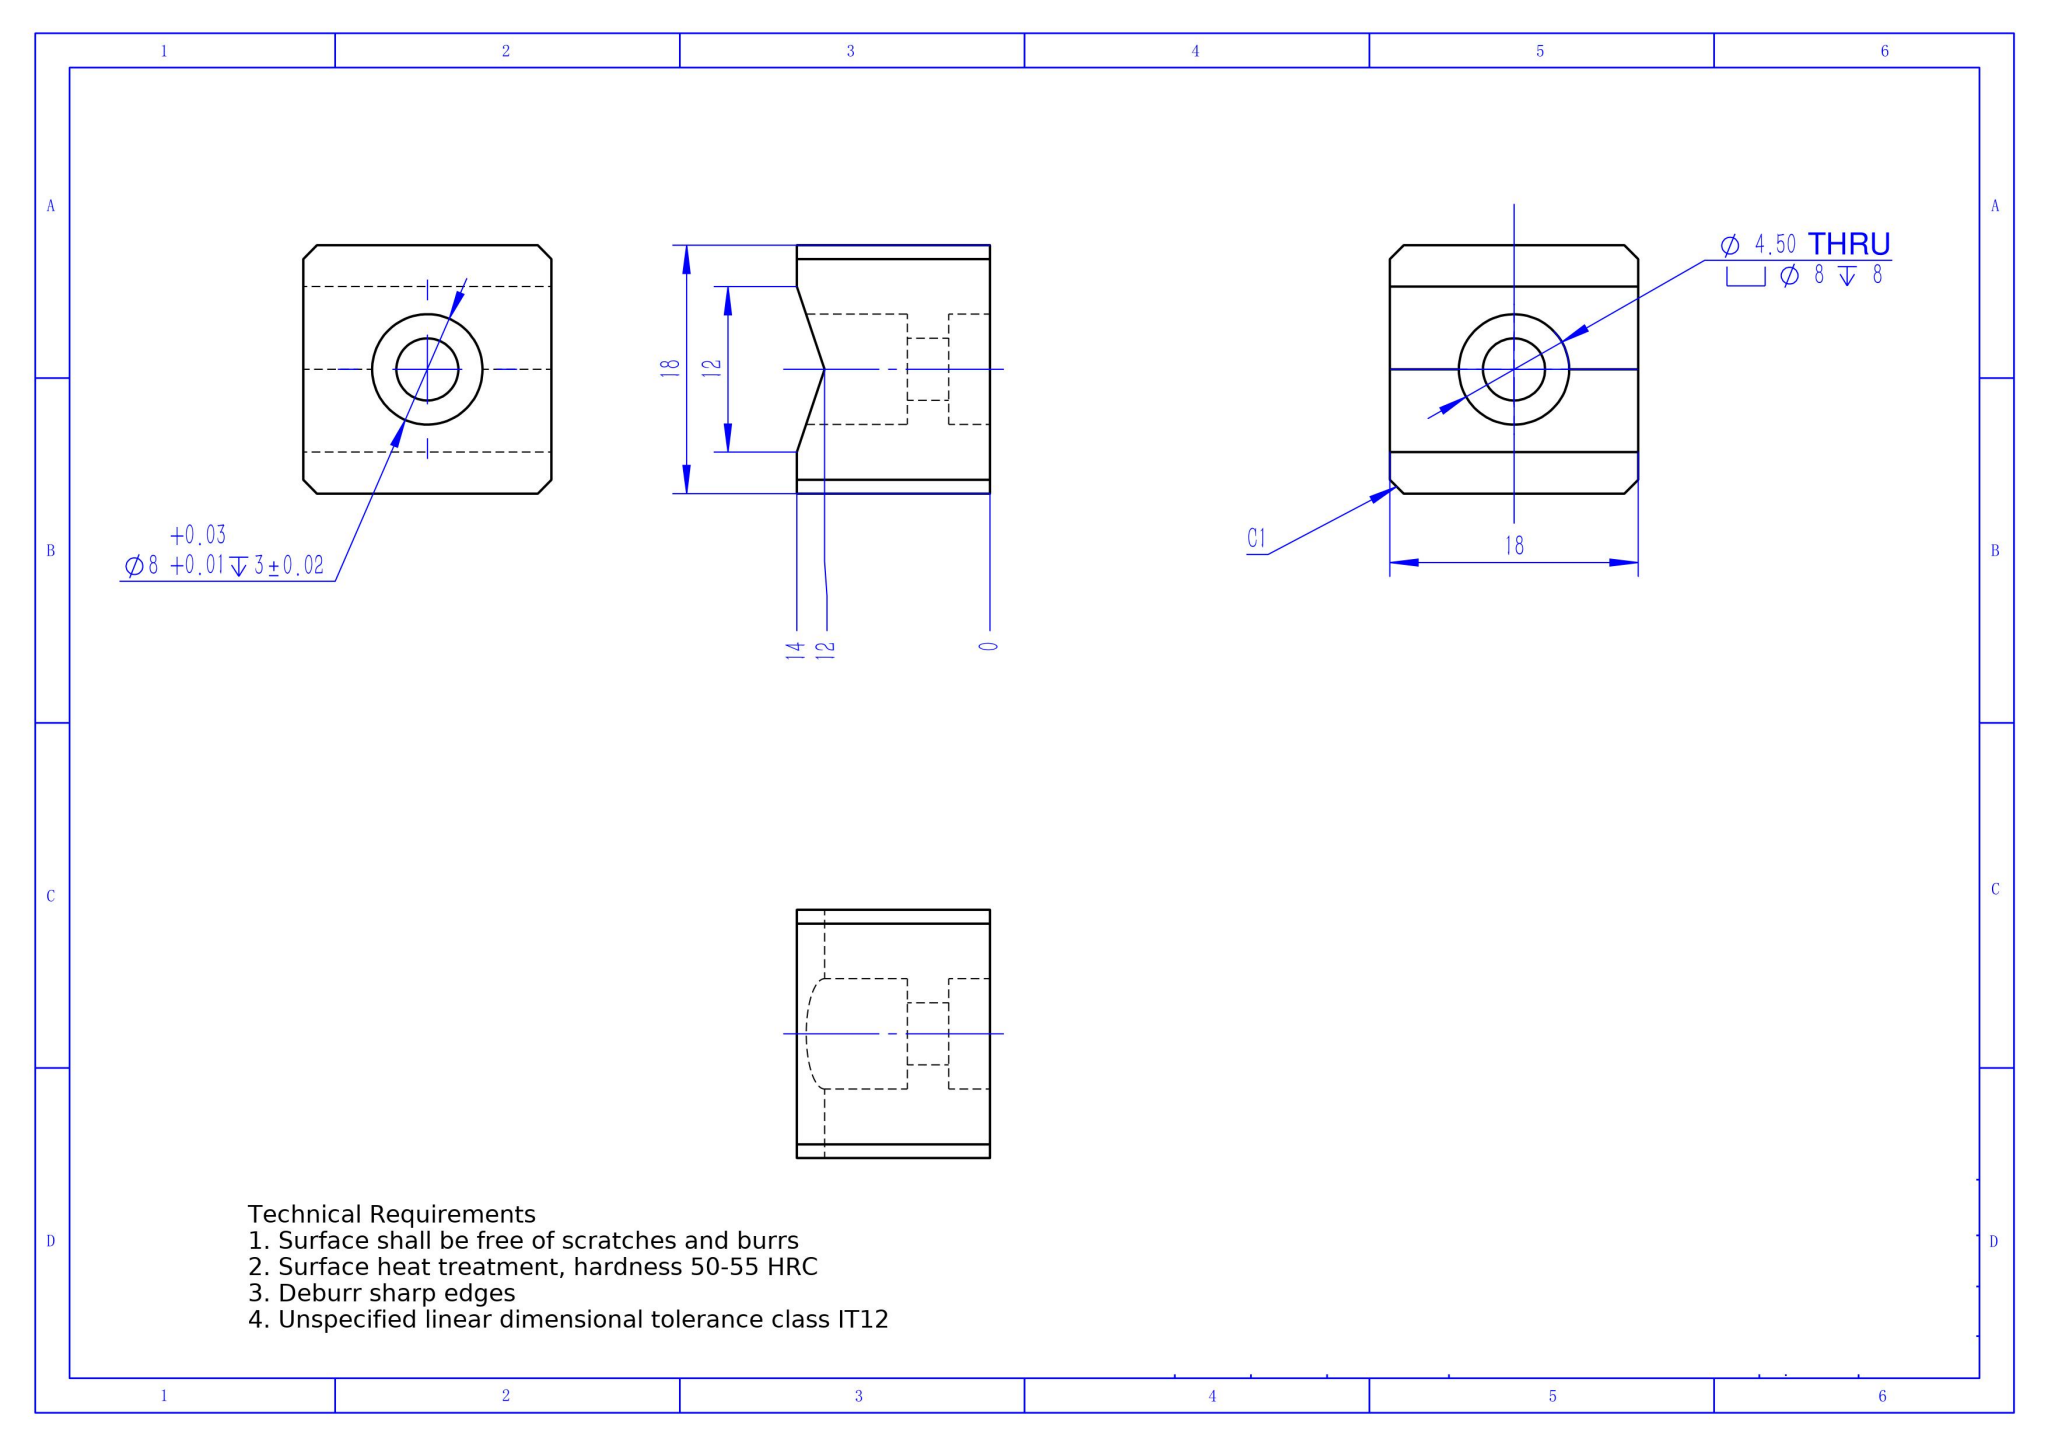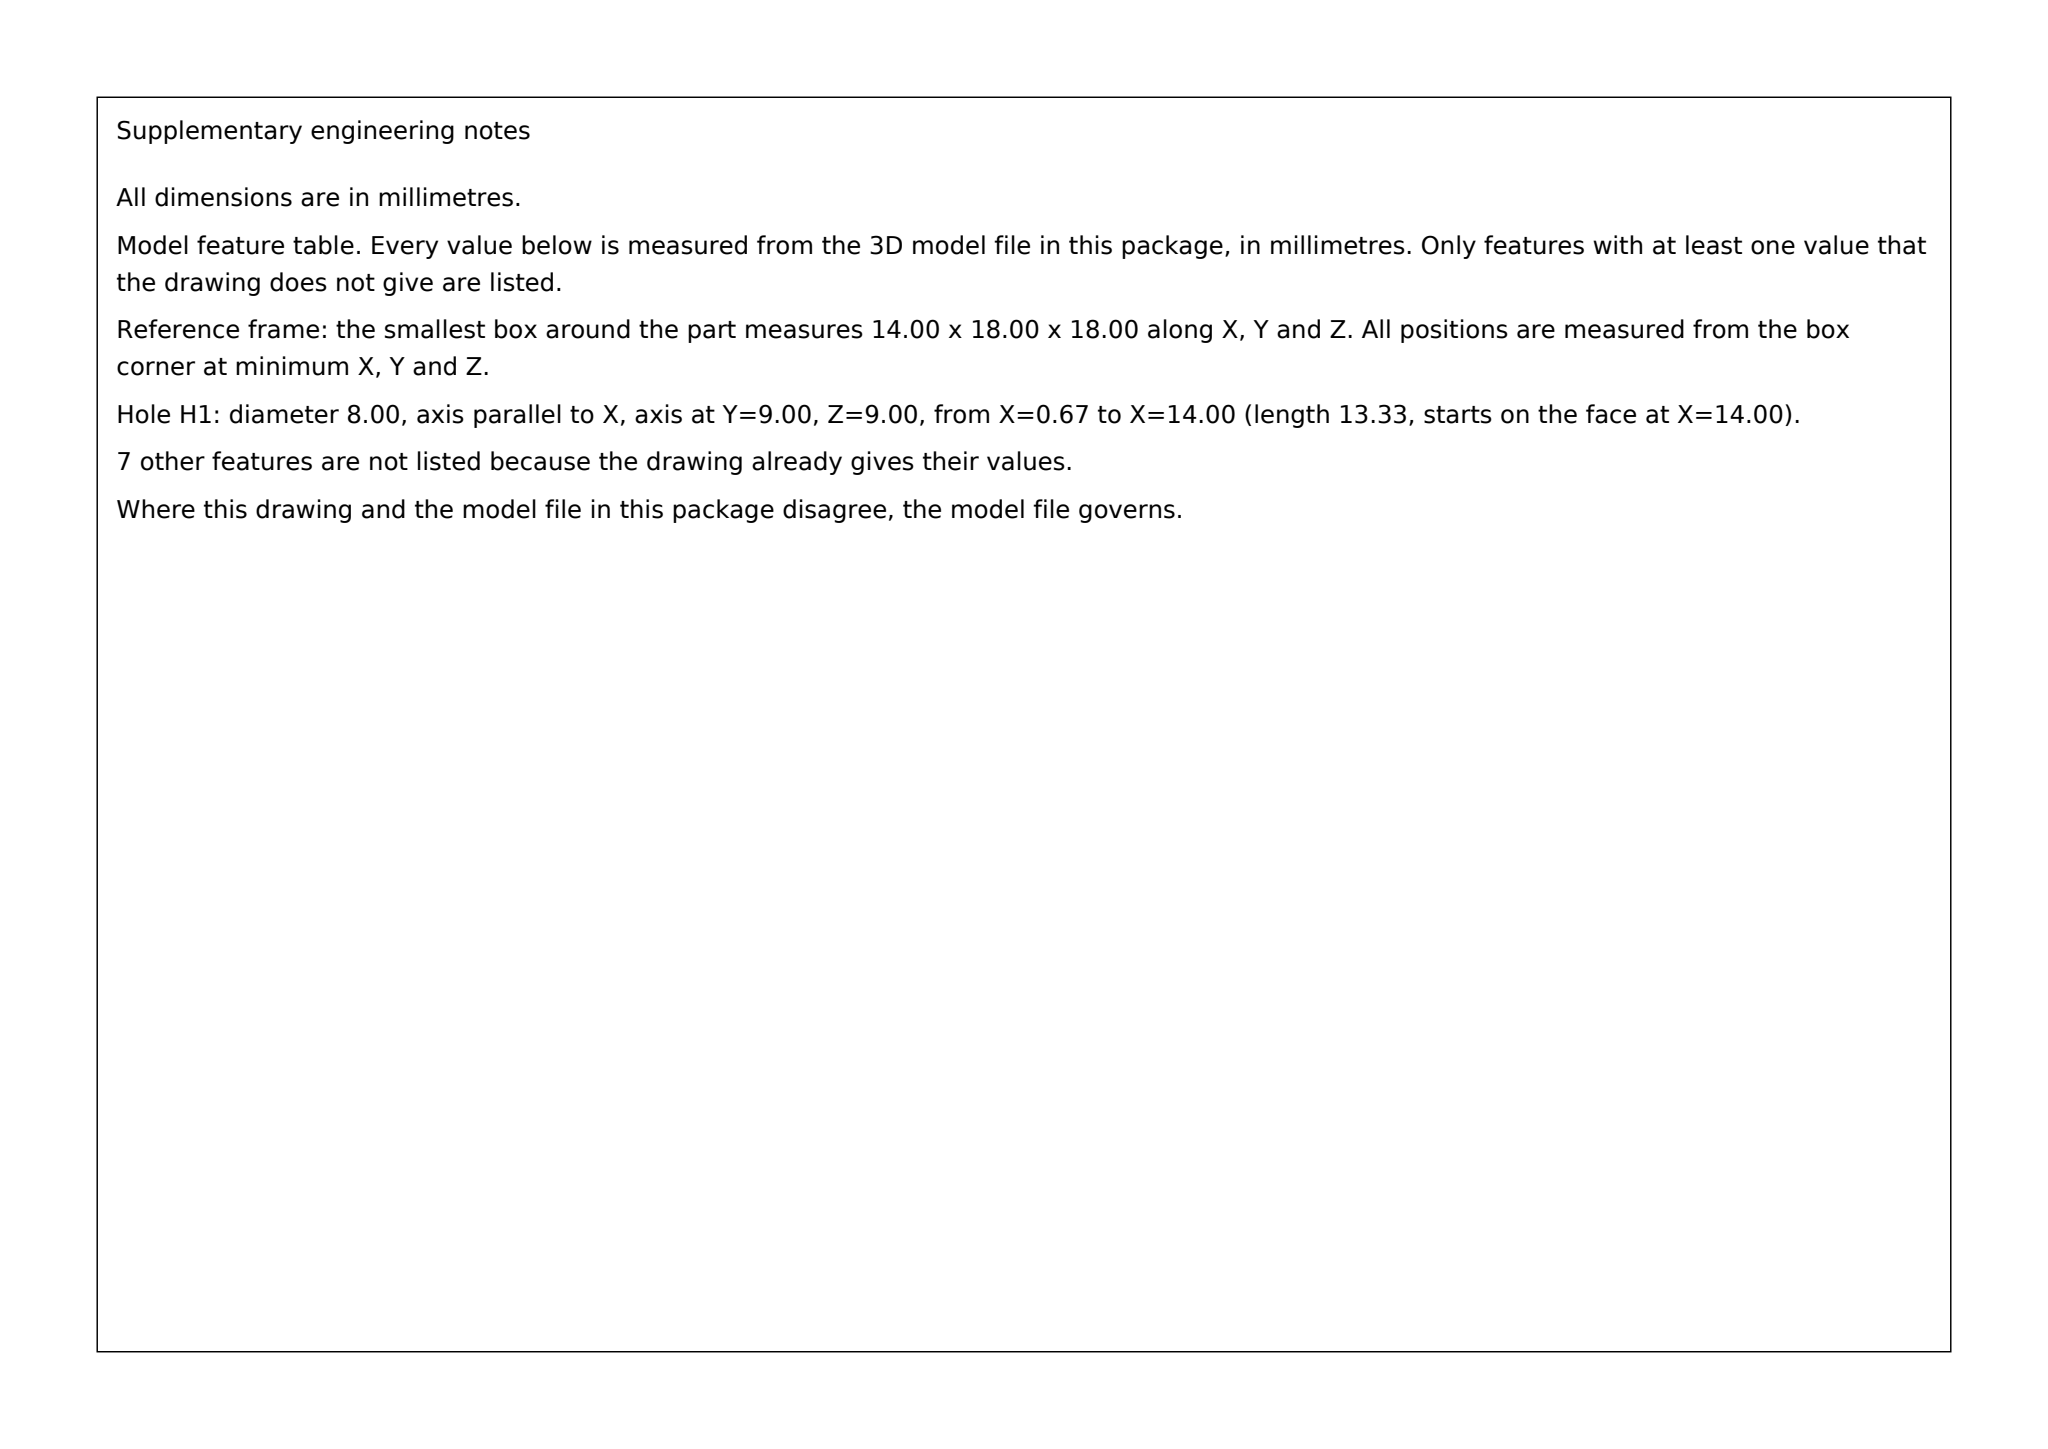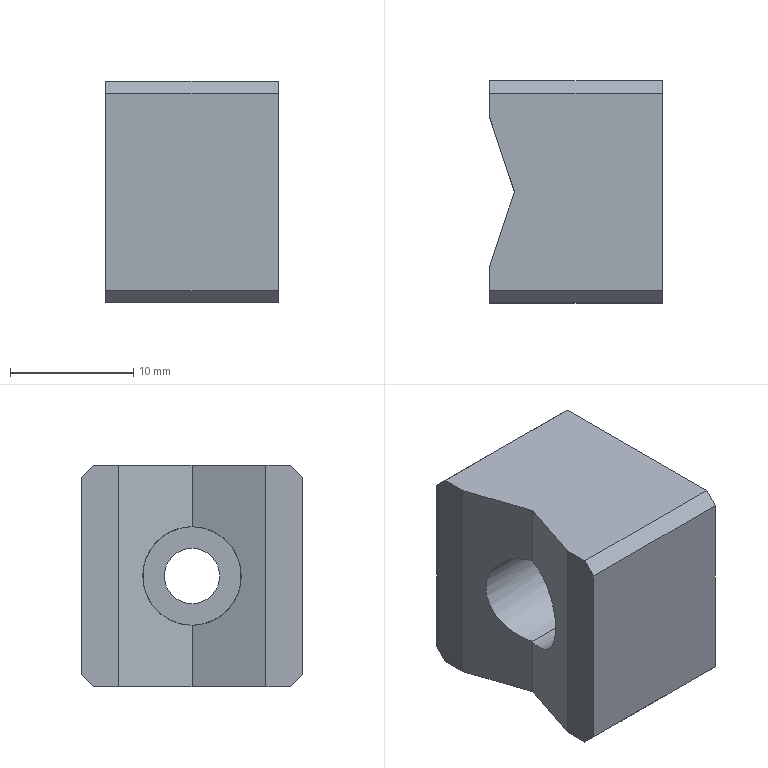Part | SolidWorks | mm | 1 solid | 21 faces | box 14 x 18 x 18 mm | volume 3763 mm3 | plane 15 | cylinder 6 | commonest cylinder face diameters 8 x4 4.5 x2
build123d program:
from build123d import *

# Parameters (mm, degrees)
BOSS_EXTRUDE1_DEPTH                               = 9
HOLE_SIZE_ACCORDING_TO_TYPE_1_OF_HEXA_D           = 4.5
HOLE_SIZE_ACCORDING_TO_TYPE_1_OF_HEXA_CBORE_D     = 8
HOLE_SIZE_ACCORDING_TO_TYPE_1_OF_HEXA_CBORE_DEPTH = 8
CUT_EXTRUDE1_START                                = -3
SKETCH4_R                                         = 4
CUT_EXTRUDE1_DEPTH                                = 3
CHAMFER1_SIZE                                     = 1


with BuildPart() as part:
    # Sketch1 → Boss-Extrude1 (new, symmetric)
    with BuildSketch(Plane.XY):
        Polygon((-14, 6), (-12, 0), (-14, -6), (-14, -9), (0, -9), (0, 9), (-14, 9), align=None)
    extrude(amount=BOSS_EXTRUDE1_DEPTH, both=True)

    # Hole Size _ according to_ type 1 of Hexa (through all)
    with Locations(Plane.ZY.offset(14)):
        with Locations((0, 0)):
            CounterBoreHole(HOLE_SIZE_ACCORDING_TO_TYPE_1_OF_HEXA_D / 2, HOLE_SIZE_ACCORDING_TO_TYPE_1_OF_HEXA_CBORE_D / 2, HOLE_SIZE_ACCORDING_TO_TYPE_1_OF_HEXA_CBORE_DEPTH)

    # Sketch4 → Cut-Extrude1 (cut)
    with BuildSketch(Plane(origin=(0, 0, 0), x_dir=(0, 0, -1), z_dir=(1, 0, 0)).offset(CUT_EXTRUDE1_START)):
        with Locations(Location((0, 0, 0), (0, 0, 180))):
            Circle(SKETCH4_R)
    extrude(amount=CUT_EXTRUDE1_DEPTH, mode=Mode.SUBTRACT)

    # Chamfer1
    chamfer1_edges = [part.edges().sort_by_distance(p)[0] for p in [
        (-7, -9, 9),
        (-7, -9, -9),
        (-7, 9, 9),
        (-7, 9, -9),
    ]]
    chamfer(chamfer1_edges, length=CHAMFER1_SIZE)


solid = part.part
STEP:
#1=CARTESIAN_POINT('',(-3.,0.,4.));
#2=VERTEX_POINT('',#1);
#3=CARTESIAN_POINT('',(-3.,0.,-4.));
#4=VERTEX_POINT('',#3);
#5=CARTESIAN_POINT('',(-3.,0.,0.));
#6=DIRECTION('',(1.,0.,0.));
#7=DIRECTION('',(0.,0.,-1.));
#8=AXIS2_PLACEMENT_3D('',#5,#6,#7);
#9=CIRCLE('',#8,4.);
#10=EDGE_CURVE('',#2,#4,#9,.T.);
#11=ORIENTED_EDGE('',*,*,#10,.F.);
#12=CARTESIAN_POINT('',(0.,0.,4.));
#13=VERTEX_POINT('',#12);
#14=CARTESIAN_POINT('',(-3.,0.,4.));
#15=DIRECTION('',(1.,0.,0.));
#16=VECTOR('',#15,1000.);
#17=LINE('',#14,#16);
#18=EDGE_CURVE('',#2,#13,#17,.T.);
#19=ORIENTED_EDGE('',*,*,#18,.T.);
#20=CARTESIAN_POINT('',(0.,0.,-4.));
#21=VERTEX_POINT('',#20);
#22=CARTESIAN_POINT('',(0.,0.,0.));
#23=DIRECTION('',(1.,0.,0.));
#24=DIRECTION('',(0.,0.,-1.));
#25=AXIS2_PLACEMENT_3D('',#22,#23,#24);
#26=CIRCLE('',#25,4.);
#27=EDGE_CURVE('',#13,#21,#26,.T.);
#28=ORIENTED_EDGE('',*,*,#27,.T.);
#29=CARTESIAN_POINT('',(-3.,0.,-4.));
#30=DIRECTION('',(1.,0.,0.));
#31=VECTOR('',#30,1000.);
#32=LINE('',#29,#31);
#33=EDGE_CURVE('',#4,#21,#32,.T.);
#34=ORIENTED_EDGE('',*,*,#33,.F.);
#35=EDGE_LOOP('',(#11,#19,#28,#34));
#36=FACE_OUTER_BOUND('',#35,.T.);
#37=CARTESIAN_POINT('',(-3.,0.,0.));
#38=DIRECTION('',(1.,0.,0.));
#39=DIRECTION('',(0.,0.,-1.));
#40=AXIS2_PLACEMENT_3D('',#37,#38,#39);
#41=CYLINDRICAL_SURFACE('',#40,4.);
#42=ADVANCED_FACE('',(#36),#41,.F.);
#43=CARTESIAN_POINT('',(-6.,0.,-4.));
#44=VERTEX_POINT('',#43);
#45=CARTESIAN_POINT('',(-6.,0.,4.));
#46=VERTEX_POINT('',#45);
#47=CARTESIAN_POINT('',(-6.,0.,0.));
#48=DIRECTION('',(-1.,0.,0.));
#49=DIRECTION('',(0.,0.,1.));
#50=AXIS2_PLACEMENT_3D('',#47,#48,#49);
#51=CIRCLE('',#50,4.);
#52=EDGE_CURVE('',#44,#46,#51,.T.);
#53=ORIENTED_EDGE('',*,*,#52,.F.);
#54=CARTESIAN_POINT('',(-12.,0.,-4.));
#55=VERTEX_POINT('',#54);
#56=CARTESIAN_POINT('',(-14.,0.,-4.));
#57=DIRECTION('',(-1.,0.,0.));
#58=VECTOR('',#57,1000.);
#59=LINE('',#56,#58);
#60=EDGE_CURVE('',#44,#55,#59,.T.);
#61=ORIENTED_EDGE('',*,*,#60,.T.);
#62=CARTESIAN_POINT('',(-12.,0.,4.));
#63=VERTEX_POINT('',#62);
#64=CARTESIAN_POINT('',(-12.,0.,4.));
#65=CARTESIAN_POINT('',(-14.667,-8.,4.));
#66=CARTESIAN_POINT('',(-14.667,-8.,-4.));
#67=CARTESIAN_POINT('',(-12.,0.,-4.));
#68=(BOUNDED_CURVE()B_SPLINE_CURVE(3,(#64,#65,#66,#67),.UNSPECIFIED.,.F.,.F.)B_SPLINE_CURVE_WITH_KNOTS((4,4),(4.712,7.854),.UNSPECIFIED.)CURVE()GEOMETRIC_REPRESENTATION_ITEM()RATIONAL_B_SPLINE_CURVE((1.,0.3333,0.3333,1.))REPRESENTATION_ITEM(''));
#69=EDGE_CURVE('',#63,#55,#68,.T.);
#70=ORIENTED_EDGE('',*,*,#69,.F.);
#71=CARTESIAN_POINT('',(-14.,0.,4.));
#72=DIRECTION('',(-1.,0.,0.));
#73=VECTOR('',#72,1000.);
#74=LINE('',#71,#73);
#75=EDGE_CURVE('',#46,#63,#74,.T.);
#76=ORIENTED_EDGE('',*,*,#75,.F.);
#77=EDGE_LOOP('',(#53,#61,#70,#76));
#78=FACE_OUTER_BOUND('',#77,.T.);
#79=CARTESIAN_POINT('',(-14.,0.,0.));
#80=DIRECTION('',(-1.,0.,0.));
#81=DIRECTION('',(0.,0.,1.));
#82=AXIS2_PLACEMENT_3D('',#79,#80,#81);
#83=CYLINDRICAL_SURFACE('',#82,4.);
#84=ADVANCED_FACE('',(#78),#83,.F.);
#85=CARTESIAN_POINT('',(-3.,0.,-2.25));
#86=VERTEX_POINT('',#85);
#87=CARTESIAN_POINT('',(-3.,0.,2.25));
#88=VERTEX_POINT('',#87);
#89=CARTESIAN_POINT('',(-3.,0.,0.));
#90=DIRECTION('',(-1.,0.,0.));
#91=DIRECTION('',(0.,0.,-1.));
#92=AXIS2_PLACEMENT_3D('',#89,#90,#91);
#93=CIRCLE('',#92,2.25);
#94=EDGE_CURVE('',#86,#88,#93,.T.);
#95=ORIENTED_EDGE('',*,*,#94,.F.);
#96=CARTESIAN_POINT('',(-6.,0.,-2.25));
#97=VERTEX_POINT('',#96);
#98=CARTESIAN_POINT('',(-14.,0.,-2.25));
#99=DIRECTION('',(-1.,0.,0.));
#100=VECTOR('',#99,1000.);
#101=LINE('',#98,#100);
#102=EDGE_CURVE('',#86,#97,#101,.T.);
#103=ORIENTED_EDGE('',*,*,#102,.T.);
#104=CARTESIAN_POINT('',(-6.,0.,2.25));
#105=VERTEX_POINT('',#104);
#106=CARTESIAN_POINT('',(-6.,0.,0.));
#107=DIRECTION('',(-1.,0.,0.));
#108=DIRECTION('',(0.,0.,1.));
#109=AXIS2_PLACEMENT_3D('',#106,#107,#108);
#110=CIRCLE('',#109,2.25);
#111=EDGE_CURVE('',#97,#105,#110,.T.);
#112=ORIENTED_EDGE('',*,*,#111,.T.);
#113=CARTESIAN_POINT('',(-14.,0.,2.25));
#114=DIRECTION('',(-1.,0.,0.));
#115=VECTOR('',#114,1000.);
#116=LINE('',#113,#115);
#117=EDGE_CURVE('',#88,#105,#116,.T.);
#118=ORIENTED_EDGE('',*,*,#117,.F.);
#119=EDGE_LOOP('',(#95,#103,#112,#118));
#120=FACE_OUTER_BOUND('',#119,.T.);
#121=CARTESIAN_POINT('',(-14.,0.,0.));
#122=DIRECTION('',(-1.,0.,0.));
#123=DIRECTION('',(0.,0.,1.));
#124=AXIS2_PLACEMENT_3D('',#121,#122,#123);
#125=CYLINDRICAL_SURFACE('',#124,2.25);
#126=ADVANCED_FACE('',(#120),#125,.F.);
#127=ORIENTED_EDGE('',*,*,#102,.F.);
#128=CARTESIAN_POINT('',(-3.,0.,0.));
#129=DIRECTION('',(-1.,0.,0.));
#130=DIRECTION('',(0.,0.,-1.));
#131=AXIS2_PLACEMENT_3D('',#128,#129,#130);
#132=CIRCLE('',#131,2.25);
#133=EDGE_CURVE('',#88,#86,#132,.T.);
#134=ORIENTED_EDGE('',*,*,#133,.F.);
#135=ORIENTED_EDGE('',*,*,#117,.T.);
#136=CARTESIAN_POINT('',(-6.,0.,0.));
#137=DIRECTION('',(-1.,0.,0.));
#138=DIRECTION('',(0.,0.,1.));
#139=AXIS2_PLACEMENT_3D('',#136,#137,#138);
#140=CIRCLE('',#139,2.25);
#141=EDGE_CURVE('',#105,#97,#140,.T.);
#142=ORIENTED_EDGE('',*,*,#141,.T.);
#143=EDGE_LOOP('',(#127,#134,#135,#142));
#144=FACE_OUTER_BOUND('',#143,.T.);
#145=CARTESIAN_POINT('',(-14.,0.,0.));
#146=DIRECTION('',(-1.,0.,0.));
#147=DIRECTION('',(0.,0.,1.));
#148=AXIS2_PLACEMENT_3D('',#145,#146,#147);
#149=CYLINDRICAL_SURFACE('',#148,2.25);
#150=ADVANCED_FACE('',(#144),#149,.F.);
#151=CARTESIAN_POINT('',(0.,0.,0.));
#152=DIRECTION('',(1.,0.,0.));
#153=DIRECTION('',(0.,0.,-1.));
#154=AXIS2_PLACEMENT_3D('',#151,#152,#153);
#155=CIRCLE('',#154,4.);
#156=EDGE_CURVE('',#21,#13,#155,.T.);
#157=ORIENTED_EDGE('',*,*,#156,.F.);
#158=ORIENTED_EDGE('',*,*,#27,.F.);
#159=EDGE_LOOP('',(#157,#158));
#160=FACE_BOUND('',#159,.T.);
#161=CARTESIAN_POINT('',(0.,-8.,9.));
#162=VERTEX_POINT('',#161);
#163=CARTESIAN_POINT('',(0.,8.,9.));
#164=VERTEX_POINT('',#163);
#165=CARTESIAN_POINT('',(0.,9.,9.));
#166=DIRECTION('',(0.,1.,0.));
#167=VECTOR('',#166,1000.);
#168=LINE('',#165,#167);
#169=EDGE_CURVE('',#162,#164,#168,.T.);
#170=ORIENTED_EDGE('',*,*,#169,.F.);
#171=CARTESIAN_POINT('',(0.,-9.,8.));
#172=VERTEX_POINT('',#171);
#173=CARTESIAN_POINT('',(0.,-8.,9.));
#174=DIRECTION('',(0.,-0.7071,-0.7071));
#175=VECTOR('',#174,1000.);
#176=LINE('',#173,#175);
#177=EDGE_CURVE('',#162,#172,#176,.T.);
#178=ORIENTED_EDGE('',*,*,#177,.T.);
#179=CARTESIAN_POINT('',(0.,-9.,-8.));
#180=VERTEX_POINT('',#179);
#181=CARTESIAN_POINT('',(0.,-9.,9.));
#182=DIRECTION('',(0.,0.,-1.));
#183=VECTOR('',#182,1000.);
#184=LINE('',#181,#183);
#185=EDGE_CURVE('',#172,#180,#184,.T.);
#186=ORIENTED_EDGE('',*,*,#185,.T.);
#187=CARTESIAN_POINT('',(0.,-8.,-9.));
#188=VERTEX_POINT('',#187);
#189=CARTESIAN_POINT('',(0.,-9.,-8.));
#190=DIRECTION('',(0.,0.7071,-0.7071));
#191=VECTOR('',#190,1000.);
#192=LINE('',#189,#191);
#193=EDGE_CURVE('',#180,#188,#192,.T.);
#194=ORIENTED_EDGE('',*,*,#193,.T.);
#195=CARTESIAN_POINT('',(0.,8.,-9.));
#196=VERTEX_POINT('',#195);
#197=CARTESIAN_POINT('',(0.,9.,-9.));
#198=DIRECTION('',(0.,1.,0.));
#199=VECTOR('',#198,1000.);
#200=LINE('',#197,#199);
#201=EDGE_CURVE('',#188,#196,#200,.T.);
#202=ORIENTED_EDGE('',*,*,#201,.T.);
#203=CARTESIAN_POINT('',(0.,9.,-8.));
#204=VERTEX_POINT('',#203);
#205=CARTESIAN_POINT('',(0.,9.,-8.));
#206=DIRECTION('',(0.,0.7071,0.7071));
#207=VECTOR('',#206,1000.);
#208=LINE('',#205,#207);
#209=EDGE_CURVE('',#196,#204,#208,.T.);
#210=ORIENTED_EDGE('',*,*,#209,.T.);
#211=CARTESIAN_POINT('',(0.,9.,8.));
#212=VERTEX_POINT('',#211);
#213=CARTESIAN_POINT('',(0.,9.,9.));
#214=DIRECTION('',(0.,0.,-1.));
#215=VECTOR('',#214,1000.);
#216=LINE('',#213,#215);
#217=EDGE_CURVE('',#212,#204,#216,.T.);
#218=ORIENTED_EDGE('',*,*,#217,.F.);
#219=CARTESIAN_POINT('',(0.,8.,9.));
#220=DIRECTION('',(0.,-0.7071,0.7071));
#221=VECTOR('',#220,1000.);
#222=LINE('',#219,#221);
#223=EDGE_CURVE('',#212,#164,#222,.T.);
#224=ORIENTED_EDGE('',*,*,#223,.T.);
#225=EDGE_LOOP('',(#170,#178,#186,#194,#202,#210,#218,#224));
#226=FACE_OUTER_BOUND('',#225,.T.);
#227=CARTESIAN_POINT('',(0.,9.,9.));
#228=DIRECTION('',(-1.,0.,0.));
#229=DIRECTION('',(0.,0.,1.));
#230=AXIS2_PLACEMENT_3D('',#227,#228,#229);
#231=PLANE('',#230);
#232=ADVANCED_FACE('',(#160,#226),#231,.F.);
#233=ORIENTED_EDGE('',*,*,#217,.T.);
#234=CARTESIAN_POINT('',(-14.,9.,-8.));
#235=VERTEX_POINT('',#234);
#236=CARTESIAN_POINT('',(-14.,9.,-8.));
#237=DIRECTION('',(-1.,0.,0.));
#238=VECTOR('',#237,1000.);
#239=LINE('',#236,#238);
#240=EDGE_CURVE('',#204,#235,#239,.T.);
#241=ORIENTED_EDGE('',*,*,#240,.T.);
#242=CARTESIAN_POINT('',(-14.,9.,8.));
#243=VERTEX_POINT('',#242);
#244=CARTESIAN_POINT('',(-14.,9.,9.));
#245=DIRECTION('',(0.,0.,-1.));
#246=VECTOR('',#245,1000.);
#247=LINE('',#244,#246);
#248=EDGE_CURVE('',#243,#235,#247,.T.);
#249=ORIENTED_EDGE('',*,*,#248,.F.);
#250=CARTESIAN_POINT('',(0.,9.,8.));
#251=DIRECTION('',(1.,-0.,0.));
#252=VECTOR('',#251,1000.);
#253=LINE('',#250,#252);
#254=EDGE_CURVE('',#243,#212,#253,.T.);
#255=ORIENTED_EDGE('',*,*,#254,.T.);
#256=EDGE_LOOP('',(#233,#241,#249,#255));
#257=FACE_OUTER_BOUND('',#256,.T.);
#258=CARTESIAN_POINT('',(0.,9.,9.));
#259=DIRECTION('',(-0.,-1.,0.));
#260=DIRECTION('',(1.,-0.,0.));
#261=AXIS2_PLACEMENT_3D('',#258,#259,#260);
#262=PLANE('',#261);
#263=ADVANCED_FACE('',(#257),#262,.F.);
#264=ORIENTED_EDGE('',*,*,#248,.T.);
#265=CARTESIAN_POINT('',(-14.,8.,-9.));
#266=VERTEX_POINT('',#265);
#267=CARTESIAN_POINT('',(-14.,9.,-8.));
#268=DIRECTION('',(-0.,-0.7071,-0.7071));
#269=VECTOR('',#268,1000.);
#270=LINE('',#267,#269);
#271=EDGE_CURVE('',#235,#266,#270,.T.);
#272=ORIENTED_EDGE('',*,*,#271,.T.);
#273=CARTESIAN_POINT('',(-14.,6.,-9.));
#274=VERTEX_POINT('',#273);
#275=CARTESIAN_POINT('',(-14.,9.,-9.));
#276=DIRECTION('',(-0.,-1.,0.));
#277=VECTOR('',#276,1000.);
#278=LINE('',#275,#277);
#279=EDGE_CURVE('',#266,#274,#278,.T.);
#280=ORIENTED_EDGE('',*,*,#279,.T.);
#281=CARTESIAN_POINT('',(-14.,6.,9.));
#282=VERTEX_POINT('',#281);
#283=CARTESIAN_POINT('',(-14.,6.,9.));
#284=DIRECTION('',(0.,0.,-1.));
#285=VECTOR('',#284,1000.);
#286=LINE('',#283,#285);
#287=EDGE_CURVE('',#282,#274,#286,.T.);
#288=ORIENTED_EDGE('',*,*,#287,.F.);
#289=CARTESIAN_POINT('',(-14.,8.,9.));
#290=VERTEX_POINT('',#289);
#291=CARTESIAN_POINT('',(-14.,9.,9.));
#292=DIRECTION('',(-0.,-1.,0.));
#293=VECTOR('',#292,1000.);
#294=LINE('',#291,#293);
#295=EDGE_CURVE('',#290,#282,#294,.T.);
#296=ORIENTED_EDGE('',*,*,#295,.F.);
#297=CARTESIAN_POINT('',(-14.,8.,9.));
#298=DIRECTION('',(0.,0.7071,-0.7071));
#299=VECTOR('',#298,1000.);
#300=LINE('',#297,#299);
#301=EDGE_CURVE('',#290,#243,#300,.T.);
#302=ORIENTED_EDGE('',*,*,#301,.T.);
#303=EDGE_LOOP('',(#264,#272,#280,#288,#296,#302));
#304=FACE_OUTER_BOUND('',#303,.T.);
#305=CARTESIAN_POINT('',(-14.,9.,9.));
#306=DIRECTION('',(1.,-0.,0.));
#307=DIRECTION('',(0.,1.,0.));
#308=AXIS2_PLACEMENT_3D('',#305,#306,#307);
#309=PLANE('',#308);
#310=ADVANCED_FACE('',(#304),#309,.F.);
#311=CARTESIAN_POINT('',(-12.,0.,-9.));
#312=VERTEX_POINT('',#311);
#313=CARTESIAN_POINT('',(-12.,0.,9.));
#314=DIRECTION('',(0.,0.,-1.));
#315=VECTOR('',#314,1000.);
#316=LINE('',#313,#315);
#317=EDGE_CURVE('',#55,#312,#316,.T.);
#318=ORIENTED_EDGE('',*,*,#317,.F.);
#319=CARTESIAN_POINT('',(-12.,0.,-4.));
#320=CARTESIAN_POINT('',(-14.667,8.,-4.));
#321=CARTESIAN_POINT('',(-14.667,8.,4.));
#322=CARTESIAN_POINT('',(-12.,0.,4.));
#323=(BOUNDED_CURVE()B_SPLINE_CURVE(3,(#319,#320,#321,#322),.UNSPECIFIED.,.F.,.F.)B_SPLINE_CURVE_WITH_KNOTS((4,4),(4.712,7.854),.UNSPECIFIED.)CURVE()GEOMETRIC_REPRESENTATION_ITEM()RATIONAL_B_SPLINE_CURVE((1.,0.3333,0.3333,1.))REPRESENTATION_ITEM(''));
#324=EDGE_CURVE('',#55,#63,#323,.T.);
#325=ORIENTED_EDGE('',*,*,#324,.T.);
#326=CARTESIAN_POINT('',(-12.,0.,9.));
#327=VERTEX_POINT('',#326);
#328=CARTESIAN_POINT('',(-12.,0.,9.));
#329=DIRECTION('',(0.,0.,-1.));
#330=VECTOR('',#329,1000.);
#331=LINE('',#328,#330);
#332=EDGE_CURVE('',#327,#63,#331,.T.);
#333=ORIENTED_EDGE('',*,*,#332,.F.);
#334=CARTESIAN_POINT('',(-14.,6.,9.));
#335=DIRECTION('',(0.3162,-0.9487,0.));
#336=VECTOR('',#335,1000.);
#337=LINE('',#334,#336);
#338=EDGE_CURVE('',#282,#327,#337,.T.);
#339=ORIENTED_EDGE('',*,*,#338,.F.);
#340=ORIENTED_EDGE('',*,*,#287,.T.);
#341=CARTESIAN_POINT('',(-14.,6.,-9.));
#342=DIRECTION('',(0.3162,-0.9487,0.));
#343=VECTOR('',#342,1000.);
#344=LINE('',#341,#343);
#345=EDGE_CURVE('',#274,#312,#344,.T.);
#346=ORIENTED_EDGE('',*,*,#345,.T.);
#347=EDGE_LOOP('',(#318,#325,#333,#339,#340,#346));
#348=FACE_OUTER_BOUND('',#347,.T.);
#349=CARTESIAN_POINT('',(-14.,6.,9.));
#350=DIRECTION('',(0.9487,0.3162,0.));
#351=DIRECTION('',(-0.3162,0.9487,0.));
#352=AXIS2_PLACEMENT_3D('',#349,#350,#351);
#353=PLANE('',#352);
#354=ADVANCED_FACE('',(#348),#353,.F.);
#355=ORIENTED_EDGE('',*,*,#332,.T.);
#356=ORIENTED_EDGE('',*,*,#69,.T.);
#357=ORIENTED_EDGE('',*,*,#317,.T.);
#358=CARTESIAN_POINT('',(-14.,-6.,-9.));
#359=VERTEX_POINT('',#358);
#360=CARTESIAN_POINT('',(-12.,0.,-9.));
#361=DIRECTION('',(-0.3162,-0.9487,0.));
#362=VECTOR('',#361,1000.);
#363=LINE('',#360,#362);
#364=EDGE_CURVE('',#312,#359,#363,.T.);
#365=ORIENTED_EDGE('',*,*,#364,.T.);
#366=CARTESIAN_POINT('',(-14.,-6.,9.));
#367=VERTEX_POINT('',#366);
#368=CARTESIAN_POINT('',(-14.,-6.,9.));
#369=DIRECTION('',(0.,0.,-1.));
#370=VECTOR('',#369,1000.);
#371=LINE('',#368,#370);
#372=EDGE_CURVE('',#367,#359,#371,.T.);
#373=ORIENTED_EDGE('',*,*,#372,.F.);
#374=CARTESIAN_POINT('',(-12.,0.,9.));
#375=DIRECTION('',(-0.3162,-0.9487,0.));
#376=VECTOR('',#375,1000.);
#377=LINE('',#374,#376);
#378=EDGE_CURVE('',#327,#367,#377,.T.);
#379=ORIENTED_EDGE('',*,*,#378,.F.);
#380=EDGE_LOOP('',(#355,#356,#357,#365,#373,#379));
#381=FACE_OUTER_BOUND('',#380,.T.);
#382=CARTESIAN_POINT('',(-12.,0.,9.));
#383=DIRECTION('',(0.9487,-0.3162,0.));
#384=DIRECTION('',(0.3162,0.9487,0.));
#385=AXIS2_PLACEMENT_3D('',#382,#383,#384);
#386=PLANE('',#385);
#387=ADVANCED_FACE('',(#381),#386,.F.);
#388=CARTESIAN_POINT('',(-14.,-9.,8.));
#389=VERTEX_POINT('',#388);
#390=CARTESIAN_POINT('',(-14.,-9.,-8.));
#391=VERTEX_POINT('',#390);
#392=CARTESIAN_POINT('',(-14.,-9.,9.));
#393=DIRECTION('',(0.,0.,-1.));
#394=VECTOR('',#393,1000.);
#395=LINE('',#392,#394);
#396=EDGE_CURVE('',#389,#391,#395,.T.);
#397=ORIENTED_EDGE('',*,*,#396,.F.);
#398=CARTESIAN_POINT('',(-14.,-8.,9.));
#399=VERTEX_POINT('',#398);
#400=CARTESIAN_POINT('',(-14.,-8.,9.));
#401=DIRECTION('',(-0.,0.7071,0.7071));
#402=VECTOR('',#401,1000.);
#403=LINE('',#400,#402);
#404=EDGE_CURVE('',#389,#399,#403,.T.);
#405=ORIENTED_EDGE('',*,*,#404,.T.);
#406=CARTESIAN_POINT('',(-14.,-6.,9.));
#407=DIRECTION('',(0.,-1.,0.));
#408=VECTOR('',#407,1000.);
#409=LINE('',#406,#408);
#410=EDGE_CURVE('',#367,#399,#409,.T.);
#411=ORIENTED_EDGE('',*,*,#410,.F.);
#412=ORIENTED_EDGE('',*,*,#372,.T.);
#413=CARTESIAN_POINT('',(-14.,-8.,-9.));
#414=VERTEX_POINT('',#413);
#415=CARTESIAN_POINT('',(-14.,-6.,-9.));
#416=DIRECTION('',(0.,-1.,0.));
#417=VECTOR('',#416,1000.);
#418=LINE('',#415,#417);
#419=EDGE_CURVE('',#359,#414,#418,.T.);
#420=ORIENTED_EDGE('',*,*,#419,.T.);
#421=CARTESIAN_POINT('',(-14.,-9.,-8.));
#422=DIRECTION('',(0.,-0.7071,0.7071));
#423=VECTOR('',#422,1000.);
#424=LINE('',#421,#423);
#425=EDGE_CURVE('',#414,#391,#424,.T.);
#426=ORIENTED_EDGE('',*,*,#425,.T.);
#427=EDGE_LOOP('',(#397,#405,#411,#412,#420,#426));
#428=FACE_OUTER_BOUND('',#427,.T.);
#429=CARTESIAN_POINT('',(-14.,-6.,9.));
#430=DIRECTION('',(1.,0.,0.));
#431=DIRECTION('',(-0.,1.,0.));
#432=AXIS2_PLACEMENT_3D('',#429,#430,#431);
#433=PLANE('',#432);
#434=ADVANCED_FACE('',(#428),#433,.F.);
#435=ORIENTED_EDGE('',*,*,#185,.F.);
#436=CARTESIAN_POINT('',(0.,-9.,8.));
#437=DIRECTION('',(-1.,-0.,0.));
#438=VECTOR('',#437,1000.);
#439=LINE('',#436,#438);
#440=EDGE_CURVE('',#172,#389,#439,.T.);
#441=ORIENTED_EDGE('',*,*,#440,.T.);
#442=ORIENTED_EDGE('',*,*,#396,.T.);
#443=CARTESIAN_POINT('',(0.,-9.,-8.));
#444=DIRECTION('',(1.,0.,0.));
#445=VECTOR('',#444,1000.);
#446=LINE('',#443,#445);
#447=EDGE_CURVE('',#391,#180,#446,.T.);
#448=ORIENTED_EDGE('',*,*,#447,.T.);
#449=EDGE_LOOP('',(#435,#441,#442,#448));
#450=FACE_OUTER_BOUND('',#449,.T.);
#451=CARTESIAN_POINT('',(0.,-9.,9.));
#452=DIRECTION('',(-0.,1.,0.));
#453=DIRECTION('',(-1.,-0.,0.));
#454=AXIS2_PLACEMENT_3D('',#451,#452,#453);
#455=PLANE('',#454);
#456=ADVANCED_FACE('',(#450),#455,.F.);
#457=ORIENTED_EDGE('',*,*,#410,.T.);
#458=CARTESIAN_POINT('',(0.,-8.,9.));
#459=DIRECTION('',(1.,0.,0.));
#460=VECTOR('',#459,1000.);
#461=LINE('',#458,#460);
#462=EDGE_CURVE('',#399,#162,#461,.T.);
#463=ORIENTED_EDGE('',*,*,#462,.T.);
#464=ORIENTED_EDGE('',*,*,#169,.T.);
#465=CARTESIAN_POINT('',(0.,8.,9.));
#466=DIRECTION('',(-1.,0.,0.));
#467=VECTOR('',#466,1000.);
#468=LINE('',#465,#467);
#469=EDGE_CURVE('',#164,#290,#468,.T.);
#470=ORIENTED_EDGE('',*,*,#469,.T.);
#471=ORIENTED_EDGE('',*,*,#295,.T.);
#472=ORIENTED_EDGE('',*,*,#338,.T.);
#473=ORIENTED_EDGE('',*,*,#378,.T.);
#474=EDGE_LOOP('',(#457,#463,#464,#470,#471,#472,#473));
#475=FACE_OUTER_BOUND('',#474,.T.);
#476=CARTESIAN_POINT('',(0.,0.,9.));
#477=DIRECTION('',(0.,0.,-1.));
#478=DIRECTION('',(-1.,0.,0.));
#479=AXIS2_PLACEMENT_3D('',#476,#477,#478);
#480=PLANE('',#479);
#481=ADVANCED_FACE('',(#475),#480,.F.);
#482=ORIENTED_EDGE('',*,*,#201,.F.);
#483=CARTESIAN_POINT('',(-14.,-8.,-9.));
#484=DIRECTION('',(-1.,-0.,0.));
#485=VECTOR('',#484,1000.);
#486=LINE('',#483,#485);
#487=EDGE_CURVE('',#188,#414,#486,.T.);
#488=ORIENTED_EDGE('',*,*,#487,.T.);
#489=ORIENTED_EDGE('',*,*,#419,.F.);
#490=ORIENTED_EDGE('',*,*,#364,.F.);
#491=ORIENTED_EDGE('',*,*,#345,.F.);
#492=ORIENTED_EDGE('',*,*,#279,.F.);
#493=CARTESIAN_POINT('',(0.,8.,-9.));
#494=DIRECTION('',(1.,-0.,0.));
#495=VECTOR('',#494,1000.);
#496=LINE('',#493,#495);
#497=EDGE_CURVE('',#266,#196,#496,.T.);
#498=ORIENTED_EDGE('',*,*,#497,.T.);
#499=EDGE_LOOP('',(#482,#488,#489,#490,#491,#492,#498));
#500=FACE_OUTER_BOUND('',#499,.T.);
#501=CARTESIAN_POINT('',(0.,0.,-9.));
#502=DIRECTION('',(0.,0.,-1.));
#503=DIRECTION('',(-1.,0.,0.));
#504=AXIS2_PLACEMENT_3D('',#501,#502,#503);
#505=PLANE('',#504);
#506=ADVANCED_FACE('',(#500),#505,.T.);
#507=ORIENTED_EDGE('',*,*,#60,.F.);
#508=CARTESIAN_POINT('',(-6.,0.,0.));
#509=DIRECTION('',(-1.,0.,0.));
#510=DIRECTION('',(0.,0.,1.));
#511=AXIS2_PLACEMENT_3D('',#508,#509,#510);
#512=CIRCLE('',#511,4.);
#513=EDGE_CURVE('',#46,#44,#512,.T.);
#514=ORIENTED_EDGE('',*,*,#513,.F.);
#515=ORIENTED_EDGE('',*,*,#75,.T.);
#516=ORIENTED_EDGE('',*,*,#324,.F.);
#517=EDGE_LOOP('',(#507,#514,#515,#516));
#518=FACE_OUTER_BOUND('',#517,.T.);
#519=CARTESIAN_POINT('',(-14.,0.,0.));
#520=DIRECTION('',(-1.,0.,0.));
#521=DIRECTION('',(0.,0.,1.));
#522=AXIS2_PLACEMENT_3D('',#519,#520,#521);
#523=CYLINDRICAL_SURFACE('',#522,4.);
#524=ADVANCED_FACE('',(#518),#523,.F.);
#525=ORIENTED_EDGE('',*,*,#141,.F.);
#526=ORIENTED_EDGE('',*,*,#111,.F.);
#527=EDGE_LOOP('',(#525,#526));
#528=FACE_BOUND('',#527,.T.);
#529=ORIENTED_EDGE('',*,*,#513,.T.);
#530=ORIENTED_EDGE('',*,*,#52,.T.);
#531=EDGE_LOOP('',(#529,#530));
#532=FACE_OUTER_BOUND('',#531,.T.);
#533=CARTESIAN_POINT('',(-6.,2.25,0.));
#534=DIRECTION('',(1.,0.,0.));
#535=DIRECTION('',(0.,0.,-1.));
#536=AXIS2_PLACEMENT_3D('',#533,#534,#535);
#537=PLANE('',#536);
#538=ADVANCED_FACE('',(#528,#532),#537,.F.);
#539=CARTESIAN_POINT('',(-3.,0.,0.));
#540=DIRECTION('',(1.,0.,0.));
#541=DIRECTION('',(0.,0.,-1.));
#542=AXIS2_PLACEMENT_3D('',#539,#540,#541);
#543=CIRCLE('',#542,4.);
#544=EDGE_CURVE('',#4,#2,#543,.T.);
#545=ORIENTED_EDGE('',*,*,#544,.T.);
#546=ORIENTED_EDGE('',*,*,#10,.T.);
#547=EDGE_LOOP('',(#545,#546));
#548=FACE_OUTER_BOUND('',#547,.T.);
#549=ORIENTED_EDGE('',*,*,#133,.T.);
#550=ORIENTED_EDGE('',*,*,#94,.T.);
#551=EDGE_LOOP('',(#549,#550));
#552=FACE_BOUND('',#551,.T.);
#553=CARTESIAN_POINT('',(-3.,0.,0.));
#554=DIRECTION('',(1.,0.,0.));
#555=DIRECTION('',(0.,0.,-1.));
#556=AXIS2_PLACEMENT_3D('',#553,#554,#555);
#557=PLANE('',#556);
#558=ADVANCED_FACE('',(#548,#552),#557,.T.);
#559=ORIENTED_EDGE('',*,*,#18,.F.);
#560=ORIENTED_EDGE('',*,*,#544,.F.);
#561=ORIENTED_EDGE('',*,*,#33,.T.);
#562=ORIENTED_EDGE('',*,*,#156,.T.);
#563=EDGE_LOOP('',(#559,#560,#561,#562));
#564=FACE_OUTER_BOUND('',#563,.T.);
#565=CARTESIAN_POINT('',(-3.,0.,0.));
#566=DIRECTION('',(1.,0.,0.));
#567=DIRECTION('',(0.,0.,-1.));
#568=AXIS2_PLACEMENT_3D('',#565,#566,#567);
#569=CYLINDRICAL_SURFACE('',#568,4.);
#570=ADVANCED_FACE('',(#564),#569,.F.);
#571=ORIENTED_EDGE('',*,*,#404,.F.);
#572=ORIENTED_EDGE('',*,*,#440,.F.);
#573=ORIENTED_EDGE('',*,*,#177,.F.);
#574=ORIENTED_EDGE('',*,*,#462,.F.);
#575=EDGE_LOOP('',(#571,#572,#573,#574));
#576=FACE_OUTER_BOUND('',#575,.T.);
#577=CARTESIAN_POINT('',(0.,-8.,9.));
#578=DIRECTION('',(-0.,0.7071,-0.7071));
#579=DIRECTION('',(1.,0.,0.));
#580=AXIS2_PLACEMENT_3D('',#577,#578,#579);
#581=PLANE('',#580);
#582=ADVANCED_FACE('',(#576),#581,.F.);
#583=ORIENTED_EDGE('',*,*,#425,.F.);
#584=ORIENTED_EDGE('',*,*,#487,.F.);
#585=ORIENTED_EDGE('',*,*,#193,.F.);
#586=ORIENTED_EDGE('',*,*,#447,.F.);
#587=EDGE_LOOP('',(#583,#584,#585,#586));
#588=FACE_OUTER_BOUND('',#587,.T.);
#589=CARTESIAN_POINT('',(0.,-9.,-8.));
#590=DIRECTION('',(0.,-0.7071,-0.7071));
#591=DIRECTION('',(-1.,-0.,0.));
#592=AXIS2_PLACEMENT_3D('',#589,#590,#591);
#593=PLANE('',#592);
#594=ADVANCED_FACE('',(#588),#593,.T.);
#595=ORIENTED_EDGE('',*,*,#209,.F.);
#596=ORIENTED_EDGE('',*,*,#497,.F.);
#597=ORIENTED_EDGE('',*,*,#271,.F.);
#598=ORIENTED_EDGE('',*,*,#240,.F.);
#599=EDGE_LOOP('',(#595,#596,#597,#598));
#600=FACE_OUTER_BOUND('',#599,.T.);
#601=CARTESIAN_POINT('',(0.,9.,-8.));
#602=DIRECTION('',(0.,0.7071,-0.7071));
#603=DIRECTION('',(1.,-0.,0.));
#604=AXIS2_PLACEMENT_3D('',#601,#602,#603);
#605=PLANE('',#604);
#606=ADVANCED_FACE('',(#600),#605,.T.);
#607=ORIENTED_EDGE('',*,*,#223,.F.);
#608=ORIENTED_EDGE('',*,*,#254,.F.);
#609=ORIENTED_EDGE('',*,*,#301,.F.);
#610=ORIENTED_EDGE('',*,*,#469,.F.);
#611=EDGE_LOOP('',(#607,#608,#609,#610));
#612=FACE_OUTER_BOUND('',#611,.T.);
#613=CARTESIAN_POINT('',(0.,8.,9.));
#614=DIRECTION('',(-0.,-0.7071,-0.7071));
#615=DIRECTION('',(-1.,0.,0.));
#616=AXIS2_PLACEMENT_3D('',#613,#614,#615);
#617=PLANE('',#616);
#618=ADVANCED_FACE('',(#612),#617,.F.);
#619=CLOSED_SHELL('',(#42,#84,#126,#150,#232,#263,#310,#354,#387,#434,#456,#481,#506,#524,#538,#558,#570,#582,#594,#606,#618));
#620=MANIFOLD_SOLID_BREP('',#619);
#621=CARTESIAN_POINT('',(0.,0.,0.));
#622=DIRECTION('',(0.,0.,1.));
#623=DIRECTION('',(1.,0.,0.));
#624=AXIS2_PLACEMENT_3D('',#621,#622,#623);
#625=(LENGTH_UNIT()NAMED_UNIT(*)SI_UNIT(.MILLI.,.METRE.));
#626=UNCERTAINTY_MEASURE_WITH_UNIT(LENGTH_MEASURE(0.00001),#625,'','');
#627=(NAMED_UNIT(*)PLANE_ANGLE_UNIT()SI_UNIT($,.RADIAN.));
#628=(NAMED_UNIT(*)SI_UNIT($,.STERADIAN.)SOLID_ANGLE_UNIT());
#629=(GEOMETRIC_REPRESENTATION_CONTEXT(3)GLOBAL_UNCERTAINTY_ASSIGNED_CONTEXT((#626))GLOBAL_UNIT_ASSIGNED_CONTEXT((#625,#627,#628))REPRESENTATION_CONTEXT('',''));
#630=ADVANCED_BREP_SHAPE_REPRESENTATION('',(#620,#624),#629);